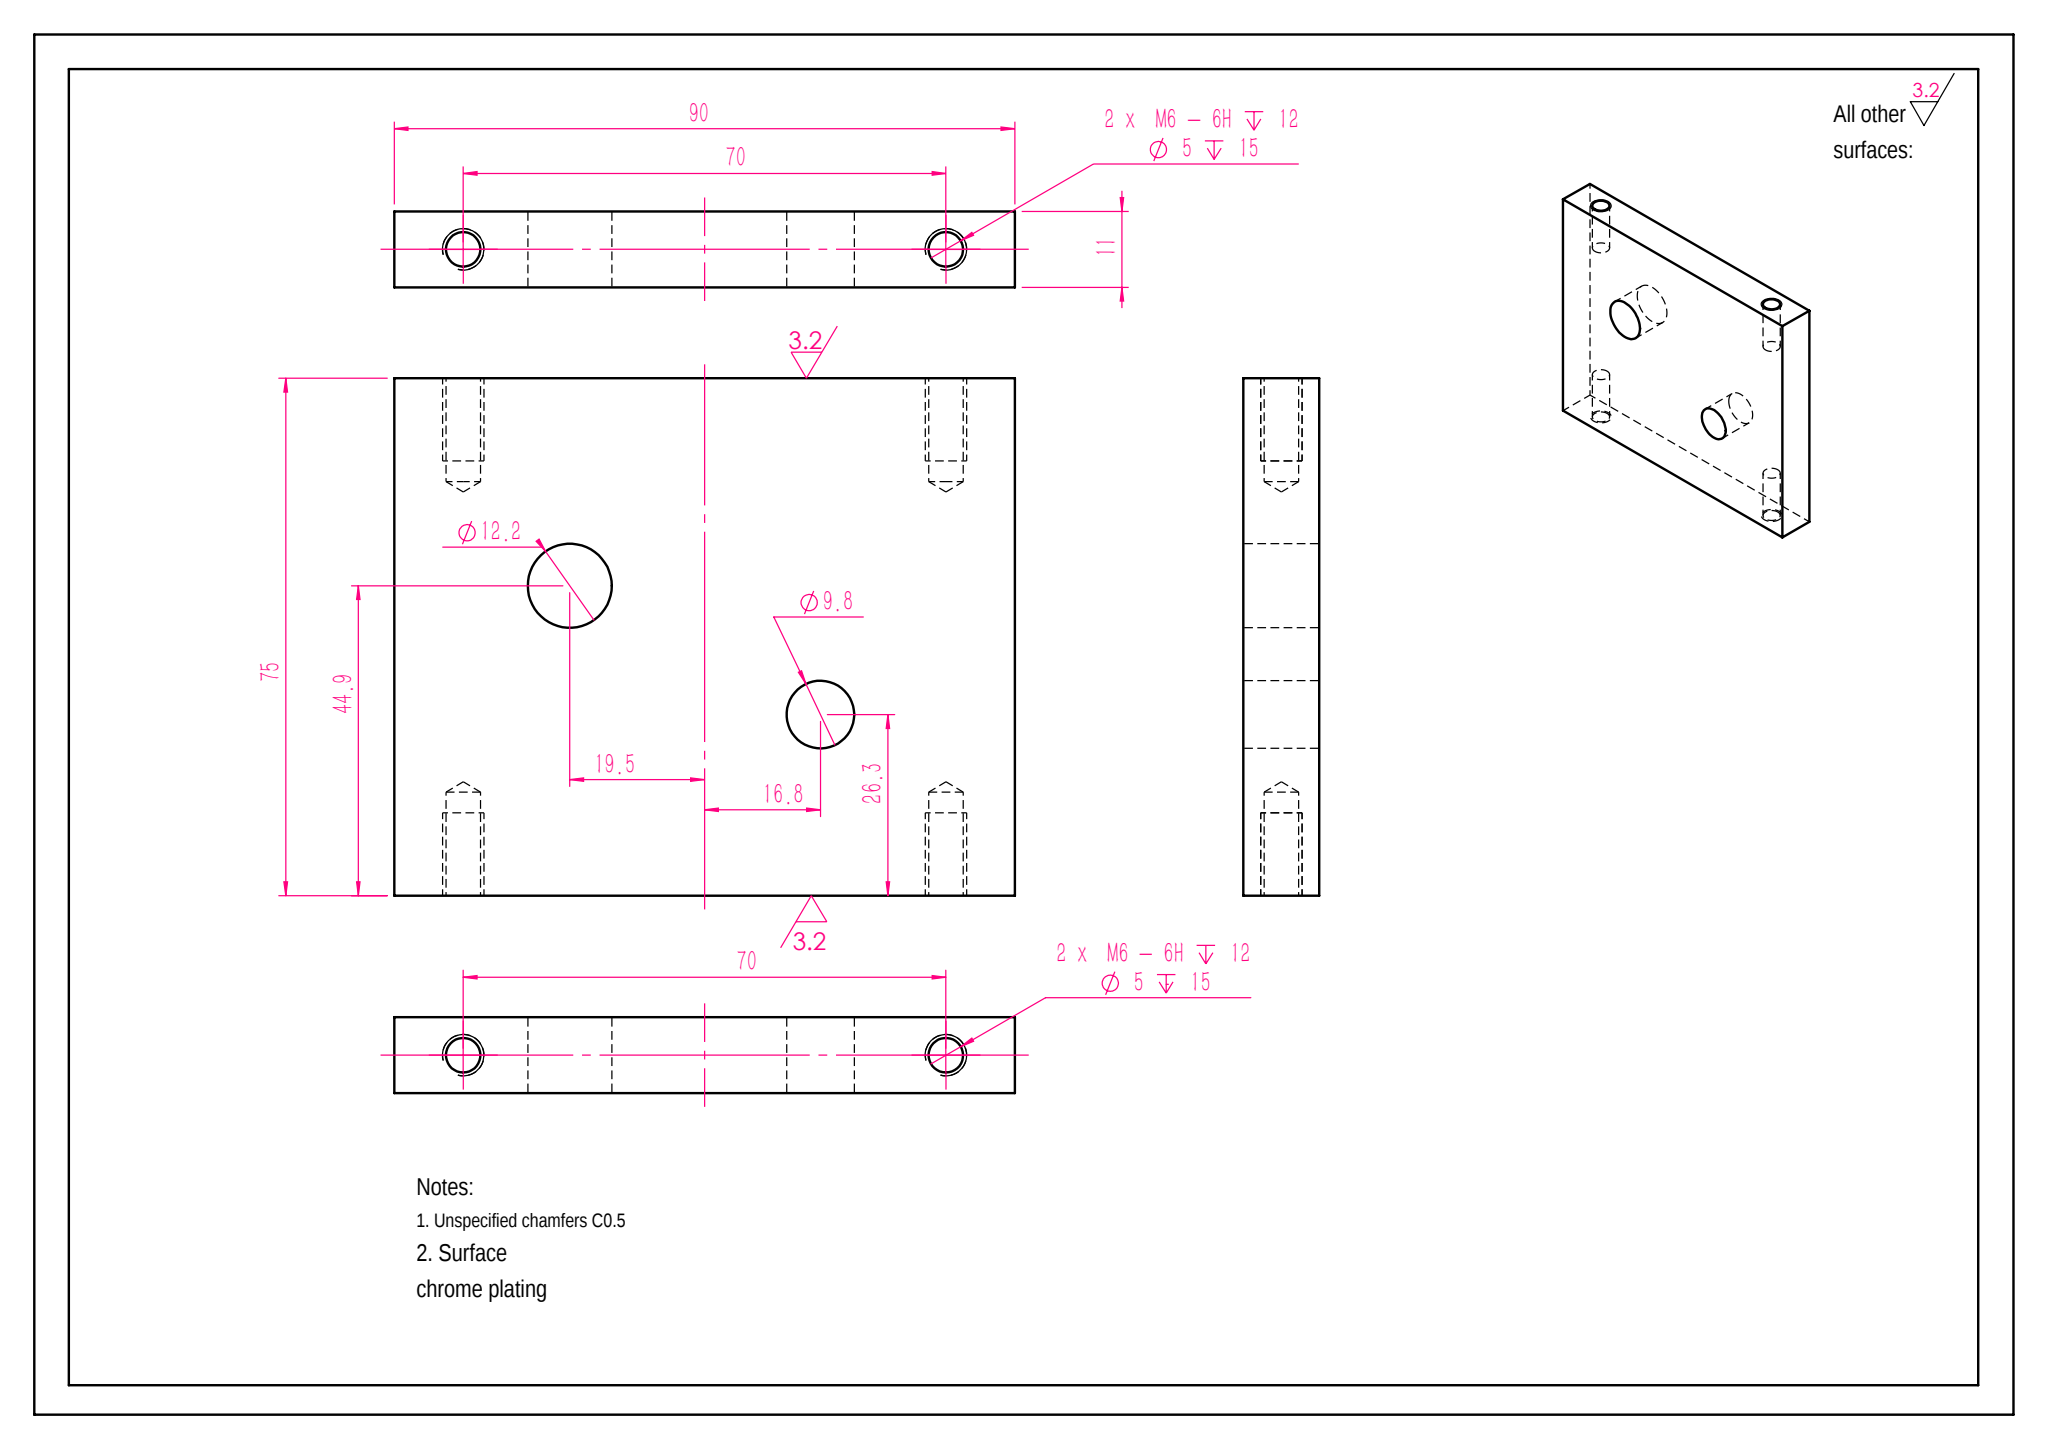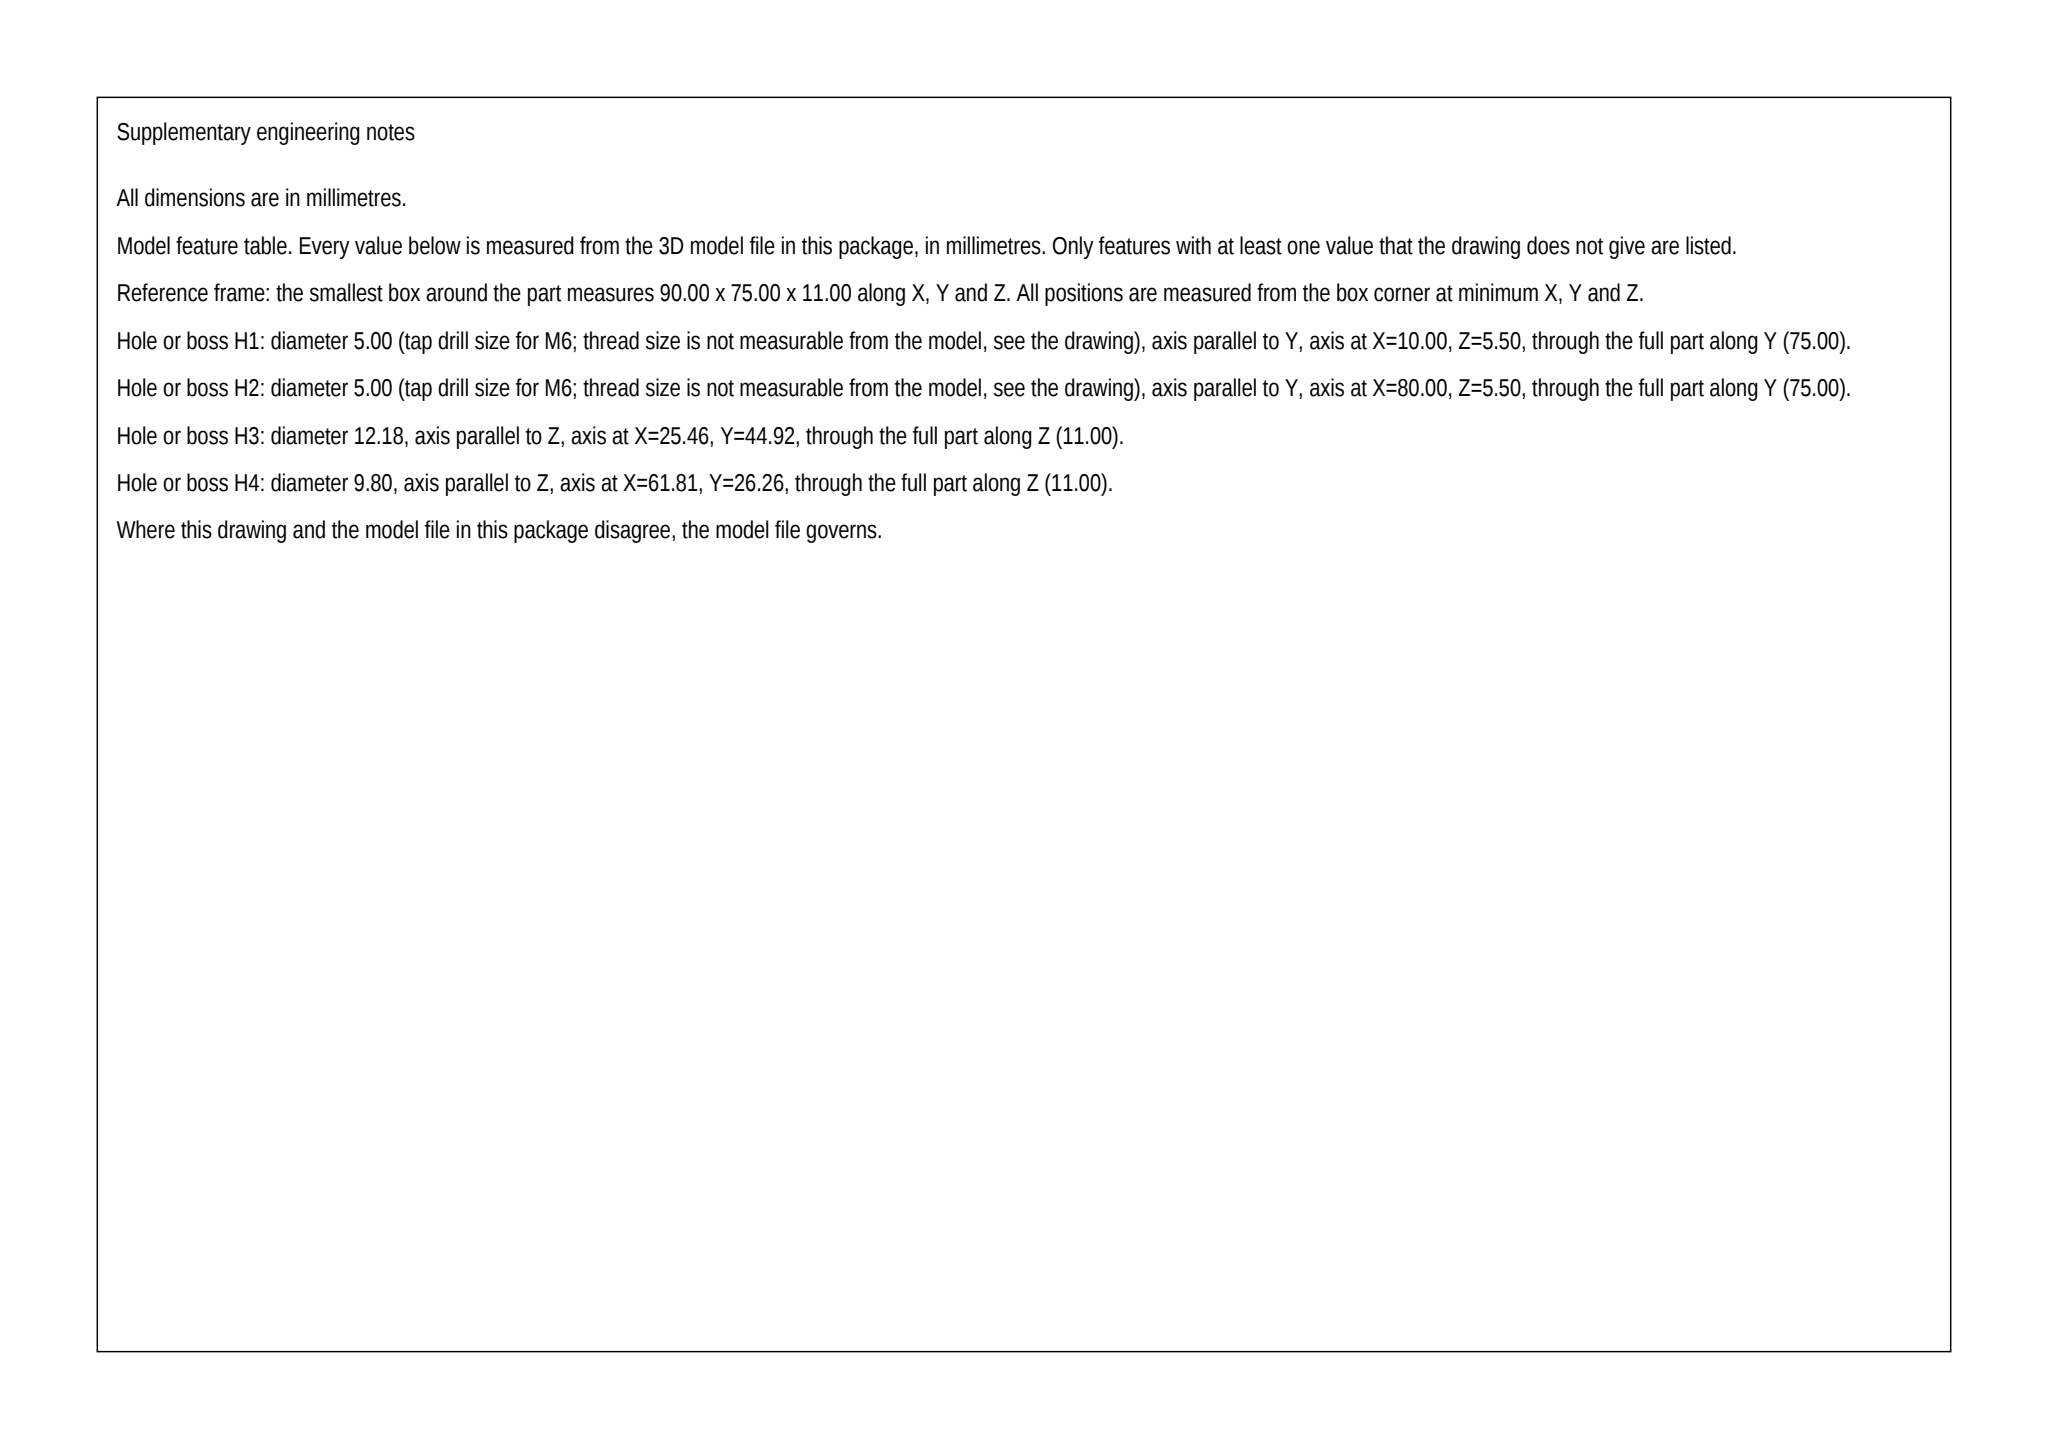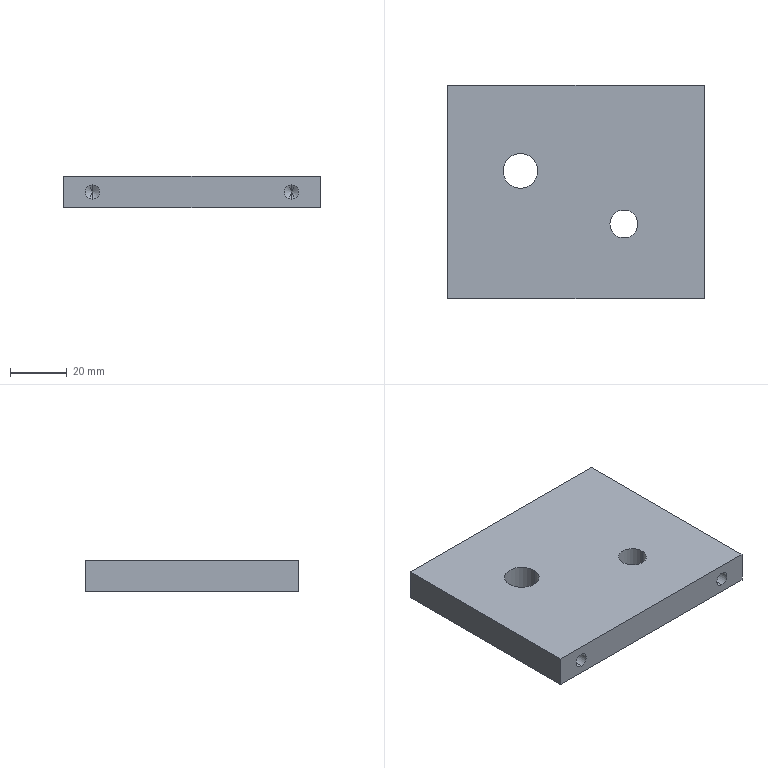Part | SolidWorks | mm | 1 solid | 26 faces | box 90 x 75 x 11 mm | volume 70920 mm3 | cylinder 12 | cone 8 | plane 6 | commonest cylinder face diameters 5 x8 12.178 x2 9.807 x2
build123d program:
from build123d import *

# Parameters (mm, degrees)
SKETCH1_W             = 90
SKETCH1_H             = 75
BOSS_EXTRUDE1_DEPTH   = 11
M6_TAPPED_HOLE1_D     = 5
M6_TAPPED_HOLE1_DEPTH = 15
M6_TAPPED_HOLE1_TIP   = 1.502
M6_TAPPED_HOLE2_D     = 5
M6_TAPPED_HOLE2_DEPTH = 15
M6_TAPPED_HOLE2_TIP   = 1.502
SKETCH6_R             = 6.089
SKETCH6_R_2           = 4.903
CUT_EXTRUDE1_DEPTH    = 80


with BuildPart() as part:
    # Sketch1 → Boss-Extrude1 (new body)
    with BuildSketch(Plane.XY):
        Rectangle(SKETCH1_W, SKETCH1_H)
    extrude(amount=BOSS_EXTRUDE1_DEPTH)

    # M6 Tapped Hole1
    with Locations(Plane(origin=(0, 37.5, 0), x_dir=(1, 0, 0), z_dir=(0, 1, 0))):
        with Locations((-35, -5.5), (35, -5.5)):
            Hole(M6_TAPPED_HOLE1_D / 2, depth=M6_TAPPED_HOLE1_DEPTH)
            with Locations((0, 0, -(M6_TAPPED_HOLE1_DEPTH + M6_TAPPED_HOLE1_TIP / 2))):  # 118° drill point
                Cone(0, M6_TAPPED_HOLE1_D / 2, M6_TAPPED_HOLE1_TIP, mode=Mode.SUBTRACT)

    # M6 Tapped Hole2
    with Locations(Plane(origin=(0, -37.5, 0), x_dir=(-1, 0, 0), z_dir=(0, -1, 0))):
        with Locations((35, -5.5), (-35, -5.5)):
            Hole(M6_TAPPED_HOLE2_D / 2, depth=M6_TAPPED_HOLE2_DEPTH)
            with Locations((0, 0, -(M6_TAPPED_HOLE2_DEPTH + M6_TAPPED_HOLE2_TIP / 2))):  # 118° drill point
                Cone(0, M6_TAPPED_HOLE2_D / 2, M6_TAPPED_HOLE2_TIP, mode=Mode.SUBTRACT)

    # Sketch6 → Cut-Extrude1 (cut)
    with BuildSketch(Plane.XY.offset(11)):
        with Locations((-19.538, 7.422)):
            Circle(SKETCH6_R)
        with Locations((16.809, -11.243)):
            Circle(SKETCH6_R_2)
    extrude(amount=-CUT_EXTRUDE1_DEPTH, mode=Mode.SUBTRACT)


solid = part.part
STEP:
#1=CARTESIAN_POINT('',(-13.449,7.422,0.));
#2=VERTEX_POINT('',#1);
#3=CARTESIAN_POINT('',(-25.627,7.422,0.));
#4=VERTEX_POINT('',#3);
#5=CARTESIAN_POINT('',(-19.538,7.422,0.));
#6=DIRECTION('',(0.,0.,-1.));
#7=DIRECTION('',(-1.,0.,0.));
#8=AXIS2_PLACEMENT_3D('',#5,#6,#7);
#9=CIRCLE('',#8,6.089);
#10=EDGE_CURVE('',#2,#4,#9,.T.);
#11=ORIENTED_EDGE('',*,*,#10,.T.);
#12=CARTESIAN_POINT('',(-25.627,7.422,11.));
#13=VERTEX_POINT('',#12);
#14=CARTESIAN_POINT('',(-25.627,7.422,-69.));
#15=DIRECTION('',(0.,0.,1.));
#16=VECTOR('',#15,1000.);
#17=LINE('',#14,#16);
#18=EDGE_CURVE('',#4,#13,#17,.T.);
#19=ORIENTED_EDGE('',*,*,#18,.T.);
#20=CARTESIAN_POINT('',(-13.449,7.422,11.));
#21=VERTEX_POINT('',#20);
#22=CARTESIAN_POINT('',(-19.538,7.422,11.));
#23=DIRECTION('',(0.,0.,1.));
#24=DIRECTION('',(1.,0.,0.));
#25=AXIS2_PLACEMENT_3D('',#22,#23,#24);
#26=CIRCLE('',#25,6.089);
#27=EDGE_CURVE('',#13,#21,#26,.T.);
#28=ORIENTED_EDGE('',*,*,#27,.T.);
#29=CARTESIAN_POINT('',(-13.449,7.422,-69.));
#30=DIRECTION('',(0.,0.,1.));
#31=VECTOR('',#30,1000.);
#32=LINE('',#29,#31);
#33=EDGE_CURVE('',#2,#21,#32,.T.);
#34=ORIENTED_EDGE('',*,*,#33,.F.);
#35=EDGE_LOOP('',(#11,#19,#28,#34));
#36=FACE_OUTER_BOUND('',#35,.T.);
#37=CARTESIAN_POINT('',(-19.538,7.422,-69.));
#38=DIRECTION('',(0.,0.,1.));
#39=DIRECTION('',(1.,0.,0.));
#40=AXIS2_PLACEMENT_3D('',#37,#38,#39);
#41=CYLINDRICAL_SURFACE('',#40,6.089);
#42=ADVANCED_FACE('',(#36),#41,.F.);
#43=CARTESIAN_POINT('',(21.713,-11.243,0.));
#44=VERTEX_POINT('',#43);
#45=CARTESIAN_POINT('',(11.906,-11.243,0.));
#46=VERTEX_POINT('',#45);
#47=CARTESIAN_POINT('',(16.809,-11.243,0.));
#48=DIRECTION('',(0.,0.,-1.));
#49=DIRECTION('',(-1.,0.,0.));
#50=AXIS2_PLACEMENT_3D('',#47,#48,#49);
#51=CIRCLE('',#50,4.903);
#52=EDGE_CURVE('',#44,#46,#51,.T.);
#53=ORIENTED_EDGE('',*,*,#52,.T.);
#54=CARTESIAN_POINT('',(11.906,-11.243,11.));
#55=VERTEX_POINT('',#54);
#56=CARTESIAN_POINT('',(11.906,-11.243,-69.));
#57=DIRECTION('',(0.,0.,1.));
#58=VECTOR('',#57,1000.);
#59=LINE('',#56,#58);
#60=EDGE_CURVE('',#46,#55,#59,.T.);
#61=ORIENTED_EDGE('',*,*,#60,.T.);
#62=CARTESIAN_POINT('',(21.713,-11.243,11.));
#63=VERTEX_POINT('',#62);
#64=CARTESIAN_POINT('',(16.809,-11.243,11.));
#65=DIRECTION('',(0.,0.,1.));
#66=DIRECTION('',(1.,0.,0.));
#67=AXIS2_PLACEMENT_3D('',#64,#65,#66);
#68=CIRCLE('',#67,4.903);
#69=EDGE_CURVE('',#55,#63,#68,.T.);
#70=ORIENTED_EDGE('',*,*,#69,.T.);
#71=CARTESIAN_POINT('',(21.713,-11.243,-69.));
#72=DIRECTION('',(0.,0.,1.));
#73=VECTOR('',#72,1000.);
#74=LINE('',#71,#73);
#75=EDGE_CURVE('',#44,#63,#74,.T.);
#76=ORIENTED_EDGE('',*,*,#75,.F.);
#77=EDGE_LOOP('',(#53,#61,#70,#76));
#78=FACE_OUTER_BOUND('',#77,.T.);
#79=CARTESIAN_POINT('',(16.809,-11.243,-69.));
#80=DIRECTION('',(0.,0.,1.));
#81=DIRECTION('',(1.,0.,0.));
#82=AXIS2_PLACEMENT_3D('',#79,#80,#81);
#83=CYLINDRICAL_SURFACE('',#82,4.903);
#84=ADVANCED_FACE('',(#78),#83,.F.);
#85=CARTESIAN_POINT('',(-35.,-22.5,8.));
#86=VERTEX_POINT('',#85);
#87=CARTESIAN_POINT('',(-35.,-22.5,3.));
#88=VERTEX_POINT('',#87);
#89=CARTESIAN_POINT('',(-35.,-22.5,5.5));
#90=DIRECTION('',(0.,-1.,0.));
#91=DIRECTION('',(0.,0.,-1.));
#92=AXIS2_PLACEMENT_3D('',#89,#90,#91);
#93=CIRCLE('',#92,2.5);
#94=EDGE_CURVE('',#86,#88,#93,.T.);
#95=ORIENTED_EDGE('',*,*,#94,.F.);
#96=CARTESIAN_POINT('',(-35.,-37.5,8.));
#97=VERTEX_POINT('',#96);
#98=CARTESIAN_POINT('',(-35.,-37.5,8.));
#99=DIRECTION('',(0.,-1.,0.));
#100=VECTOR('',#99,1000.);
#101=LINE('',#98,#100);
#102=EDGE_CURVE('',#86,#97,#101,.T.);
#103=ORIENTED_EDGE('',*,*,#102,.T.);
#104=CARTESIAN_POINT('',(-35.,-37.5,3.));
#105=VERTEX_POINT('',#104);
#106=CARTESIAN_POINT('',(-35.,-37.5,5.5));
#107=DIRECTION('',(0.,-1.,0.));
#108=DIRECTION('',(0.,0.,-1.));
#109=AXIS2_PLACEMENT_3D('',#106,#107,#108);
#110=CIRCLE('',#109,2.5);
#111=EDGE_CURVE('',#97,#105,#110,.T.);
#112=ORIENTED_EDGE('',*,*,#111,.T.);
#113=CARTESIAN_POINT('',(-35.,-37.5,3.));
#114=DIRECTION('',(0.,-1.,0.));
#115=VECTOR('',#114,1000.);
#116=LINE('',#113,#115);
#117=EDGE_CURVE('',#88,#105,#116,.T.);
#118=ORIENTED_EDGE('',*,*,#117,.F.);
#119=EDGE_LOOP('',(#95,#103,#112,#118));
#120=FACE_OUTER_BOUND('',#119,.T.);
#121=CARTESIAN_POINT('',(-35.,-37.5,5.5));
#122=DIRECTION('',(0.,-1.,0.));
#123=DIRECTION('',(0.,0.,-1.));
#124=AXIS2_PLACEMENT_3D('',#121,#122,#123);
#125=CYLINDRICAL_SURFACE('',#124,2.5);
#126=ADVANCED_FACE('',(#120),#125,.F.);
#127=CARTESIAN_POINT('',(-35.,-20.998,5.5));
#128=VERTEX_POINT('',#127);
#129=CARTESIAN_POINT('',(-35.,-22.5,3.));
#130=DIRECTION('',(0.,-0.515,-0.8572));
#131=VECTOR('',#130,1000.);
#132=LINE('',#129,#131);
#133=EDGE_CURVE('',#128,#88,#132,.T.);
#134=ORIENTED_EDGE('',*,*,#133,.F.);
#135=CARTESIAN_POINT('',(-35.,-22.5,8.));
#136=DIRECTION('',(0.,-0.515,0.8572));
#137=VECTOR('',#136,1000.);
#138=LINE('',#135,#137);
#139=EDGE_CURVE('',#128,#86,#138,.T.);
#140=ORIENTED_EDGE('',*,*,#139,.T.);
#141=ORIENTED_EDGE('',*,*,#94,.T.);
#142=EDGE_LOOP('',(#134,#140,#141));
#143=FACE_OUTER_BOUND('',#142,.T.);
#144=CARTESIAN_POINT('',(-35.,-22.5,5.5));
#145=DIRECTION('',(0.,-1.,0.));
#146=DIRECTION('',(0.,0.,-1.));
#147=AXIS2_PLACEMENT_3D('',#144,#145,#146);
#148=CONICAL_SURFACE('',#147,2.5,1.03);
#149=ADVANCED_FACE('',(#143),#148,.F.);
#150=CARTESIAN_POINT('',(35.,-22.5,8.));
#151=VERTEX_POINT('',#150);
#152=CARTESIAN_POINT('',(35.,-22.5,3.));
#153=VERTEX_POINT('',#152);
#154=CARTESIAN_POINT('',(35.,-22.5,5.5));
#155=DIRECTION('',(0.,-1.,0.));
#156=DIRECTION('',(0.,0.,-1.));
#157=AXIS2_PLACEMENT_3D('',#154,#155,#156);
#158=CIRCLE('',#157,2.5);
#159=EDGE_CURVE('',#151,#153,#158,.T.);
#160=ORIENTED_EDGE('',*,*,#159,.F.);
#161=CARTESIAN_POINT('',(35.,-37.5,8.));
#162=VERTEX_POINT('',#161);
#163=CARTESIAN_POINT('',(35.,-37.5,8.));
#164=DIRECTION('',(0.,-1.,0.));
#165=VECTOR('',#164,1000.);
#166=LINE('',#163,#165);
#167=EDGE_CURVE('',#151,#162,#166,.T.);
#168=ORIENTED_EDGE('',*,*,#167,.T.);
#169=CARTESIAN_POINT('',(35.,-37.5,3.));
#170=VERTEX_POINT('',#169);
#171=CARTESIAN_POINT('',(35.,-37.5,5.5));
#172=DIRECTION('',(0.,-1.,0.));
#173=DIRECTION('',(0.,0.,-1.));
#174=AXIS2_PLACEMENT_3D('',#171,#172,#173);
#175=CIRCLE('',#174,2.5);
#176=EDGE_CURVE('',#162,#170,#175,.T.);
#177=ORIENTED_EDGE('',*,*,#176,.T.);
#178=CARTESIAN_POINT('',(35.,-37.5,3.));
#179=DIRECTION('',(0.,-1.,0.));
#180=VECTOR('',#179,1000.);
#181=LINE('',#178,#180);
#182=EDGE_CURVE('',#153,#170,#181,.T.);
#183=ORIENTED_EDGE('',*,*,#182,.F.);
#184=EDGE_LOOP('',(#160,#168,#177,#183));
#185=FACE_OUTER_BOUND('',#184,.T.);
#186=CARTESIAN_POINT('',(35.,-37.5,5.5));
#187=DIRECTION('',(0.,-1.,0.));
#188=DIRECTION('',(0.,0.,-1.));
#189=AXIS2_PLACEMENT_3D('',#186,#187,#188);
#190=CYLINDRICAL_SURFACE('',#189,2.5);
#191=ADVANCED_FACE('',(#185),#190,.F.);
#192=CARTESIAN_POINT('',(35.,-20.998,5.5));
#193=VERTEX_POINT('',#192);
#194=CARTESIAN_POINT('',(35.,-22.5,3.));
#195=DIRECTION('',(0.,-0.515,-0.8572));
#196=VECTOR('',#195,1000.);
#197=LINE('',#194,#196);
#198=EDGE_CURVE('',#193,#153,#197,.T.);
#199=ORIENTED_EDGE('',*,*,#198,.F.);
#200=CARTESIAN_POINT('',(35.,-22.5,8.));
#201=DIRECTION('',(0.,-0.515,0.8572));
#202=VECTOR('',#201,1000.);
#203=LINE('',#200,#202);
#204=EDGE_CURVE('',#193,#151,#203,.T.);
#205=ORIENTED_EDGE('',*,*,#204,.T.);
#206=ORIENTED_EDGE('',*,*,#159,.T.);
#207=EDGE_LOOP('',(#199,#205,#206));
#208=FACE_OUTER_BOUND('',#207,.T.);
#209=CARTESIAN_POINT('',(35.,-22.5,5.5));
#210=DIRECTION('',(0.,-1.,0.));
#211=DIRECTION('',(0.,0.,-1.));
#212=AXIS2_PLACEMENT_3D('',#209,#210,#211);
#213=CONICAL_SURFACE('',#212,2.5,1.03);
#214=ADVANCED_FACE('',(#208),#213,.F.);
#215=CARTESIAN_POINT('',(-35.,22.5,3.));
#216=VERTEX_POINT('',#215);
#217=CARTESIAN_POINT('',(-35.,22.5,8.));
#218=VERTEX_POINT('',#217);
#219=CARTESIAN_POINT('',(-35.,22.5,5.5));
#220=DIRECTION('',(0.,1.,0.));
#221=DIRECTION('',(0.,0.,1.));
#222=AXIS2_PLACEMENT_3D('',#219,#220,#221);
#223=CIRCLE('',#222,2.5);
#224=EDGE_CURVE('',#216,#218,#223,.T.);
#225=ORIENTED_EDGE('',*,*,#224,.F.);
#226=CARTESIAN_POINT('',(-35.,37.5,3.));
#227=VERTEX_POINT('',#226);
#228=CARTESIAN_POINT('',(-35.,37.5,3.));
#229=DIRECTION('',(0.,1.,0.));
#230=VECTOR('',#229,1000.);
#231=LINE('',#228,#230);
#232=EDGE_CURVE('',#216,#227,#231,.T.);
#233=ORIENTED_EDGE('',*,*,#232,.T.);
#234=CARTESIAN_POINT('',(-35.,37.5,8.));
#235=VERTEX_POINT('',#234);
#236=CARTESIAN_POINT('',(-35.,37.5,5.5));
#237=DIRECTION('',(0.,1.,0.));
#238=DIRECTION('',(0.,0.,1.));
#239=AXIS2_PLACEMENT_3D('',#236,#237,#238);
#240=CIRCLE('',#239,2.5);
#241=EDGE_CURVE('',#227,#235,#240,.T.);
#242=ORIENTED_EDGE('',*,*,#241,.T.);
#243=CARTESIAN_POINT('',(-35.,37.5,8.));
#244=DIRECTION('',(0.,1.,0.));
#245=VECTOR('',#244,1000.);
#246=LINE('',#243,#245);
#247=EDGE_CURVE('',#218,#235,#246,.T.);
#248=ORIENTED_EDGE('',*,*,#247,.F.);
#249=EDGE_LOOP('',(#225,#233,#242,#248));
#250=FACE_OUTER_BOUND('',#249,.T.);
#251=CARTESIAN_POINT('',(-35.,37.5,5.5));
#252=DIRECTION('',(0.,1.,0.));
#253=DIRECTION('',(0.,0.,1.));
#254=AXIS2_PLACEMENT_3D('',#251,#252,#253);
#255=CYLINDRICAL_SURFACE('',#254,2.5);
#256=ADVANCED_FACE('',(#250),#255,.F.);
#257=CARTESIAN_POINT('',(-35.,20.998,5.5));
#258=VERTEX_POINT('',#257);
#259=CARTESIAN_POINT('',(-35.,22.5,8.));
#260=DIRECTION('',(0.,0.515,0.8572));
#261=VECTOR('',#260,1000.);
#262=LINE('',#259,#261);
#263=EDGE_CURVE('',#258,#218,#262,.T.);
#264=ORIENTED_EDGE('',*,*,#263,.F.);
#265=CARTESIAN_POINT('',(-35.,22.5,3.));
#266=DIRECTION('',(0.,0.515,-0.8572));
#267=VECTOR('',#266,1000.);
#268=LINE('',#265,#267);
#269=EDGE_CURVE('',#258,#216,#268,.T.);
#270=ORIENTED_EDGE('',*,*,#269,.T.);
#271=ORIENTED_EDGE('',*,*,#224,.T.);
#272=EDGE_LOOP('',(#264,#270,#271));
#273=FACE_OUTER_BOUND('',#272,.T.);
#274=CARTESIAN_POINT('',(-35.,22.5,5.5));
#275=DIRECTION('',(0.,1.,0.));
#276=DIRECTION('',(0.,0.,1.));
#277=AXIS2_PLACEMENT_3D('',#274,#275,#276);
#278=CONICAL_SURFACE('',#277,2.5,1.03);
#279=ADVANCED_FACE('',(#273),#278,.F.);
#280=CARTESIAN_POINT('',(35.,22.5,3.));
#281=VERTEX_POINT('',#280);
#282=CARTESIAN_POINT('',(35.,22.5,8.));
#283=VERTEX_POINT('',#282);
#284=CARTESIAN_POINT('',(35.,22.5,5.5));
#285=DIRECTION('',(0.,1.,0.));
#286=DIRECTION('',(0.,0.,1.));
#287=AXIS2_PLACEMENT_3D('',#284,#285,#286);
#288=CIRCLE('',#287,2.5);
#289=EDGE_CURVE('',#281,#283,#288,.T.);
#290=ORIENTED_EDGE('',*,*,#289,.F.);
#291=CARTESIAN_POINT('',(35.,37.5,3.));
#292=VERTEX_POINT('',#291);
#293=CARTESIAN_POINT('',(35.,37.5,3.));
#294=DIRECTION('',(0.,1.,0.));
#295=VECTOR('',#294,1000.);
#296=LINE('',#293,#295);
#297=EDGE_CURVE('',#281,#292,#296,.T.);
#298=ORIENTED_EDGE('',*,*,#297,.T.);
#299=CARTESIAN_POINT('',(35.,37.5,8.));
#300=VERTEX_POINT('',#299);
#301=CARTESIAN_POINT('',(35.,37.5,5.5));
#302=DIRECTION('',(0.,1.,0.));
#303=DIRECTION('',(0.,0.,1.));
#304=AXIS2_PLACEMENT_3D('',#301,#302,#303);
#305=CIRCLE('',#304,2.5);
#306=EDGE_CURVE('',#292,#300,#305,.T.);
#307=ORIENTED_EDGE('',*,*,#306,.T.);
#308=CARTESIAN_POINT('',(35.,37.5,8.));
#309=DIRECTION('',(0.,1.,0.));
#310=VECTOR('',#309,1000.);
#311=LINE('',#308,#310);
#312=EDGE_CURVE('',#283,#300,#311,.T.);
#313=ORIENTED_EDGE('',*,*,#312,.F.);
#314=EDGE_LOOP('',(#290,#298,#307,#313));
#315=FACE_OUTER_BOUND('',#314,.T.);
#316=CARTESIAN_POINT('',(35.,37.5,5.5));
#317=DIRECTION('',(0.,1.,0.));
#318=DIRECTION('',(0.,0.,1.));
#319=AXIS2_PLACEMENT_3D('',#316,#317,#318);
#320=CYLINDRICAL_SURFACE('',#319,2.5);
#321=ADVANCED_FACE('',(#315),#320,.F.);
#322=CARTESIAN_POINT('',(35.,20.998,5.5));
#323=VERTEX_POINT('',#322);
#324=CARTESIAN_POINT('',(35.,22.5,8.));
#325=DIRECTION('',(0.,0.515,0.8572));
#326=VECTOR('',#325,1000.);
#327=LINE('',#324,#326);
#328=EDGE_CURVE('',#323,#283,#327,.T.);
#329=ORIENTED_EDGE('',*,*,#328,.F.);
#330=CARTESIAN_POINT('',(35.,22.5,3.));
#331=DIRECTION('',(0.,0.515,-0.8572));
#332=VECTOR('',#331,1000.);
#333=LINE('',#330,#332);
#334=EDGE_CURVE('',#323,#281,#333,.T.);
#335=ORIENTED_EDGE('',*,*,#334,.T.);
#336=ORIENTED_EDGE('',*,*,#289,.T.);
#337=EDGE_LOOP('',(#329,#335,#336));
#338=FACE_OUTER_BOUND('',#337,.T.);
#339=CARTESIAN_POINT('',(35.,22.5,5.5));
#340=DIRECTION('',(0.,1.,0.));
#341=DIRECTION('',(0.,0.,1.));
#342=AXIS2_PLACEMENT_3D('',#339,#340,#341);
#343=CONICAL_SURFACE('',#342,2.5,1.03);
#344=ADVANCED_FACE('',(#338),#343,.F.);
#345=CARTESIAN_POINT('',(45.,-37.5,0.));
#346=VERTEX_POINT('',#345);
#347=CARTESIAN_POINT('',(45.,37.5,0.));
#348=VERTEX_POINT('',#347);
#349=CARTESIAN_POINT('',(45.,-37.5,0.));
#350=DIRECTION('',(0.,1.,0.));
#351=VECTOR('',#350,1000.);
#352=LINE('',#349,#351);
#353=EDGE_CURVE('',#346,#348,#352,.T.);
#354=ORIENTED_EDGE('',*,*,#353,.T.);
#355=CARTESIAN_POINT('',(45.,37.5,11.));
#356=VERTEX_POINT('',#355);
#357=CARTESIAN_POINT('',(45.,37.5,11.));
#358=DIRECTION('',(0.,0.,-1.));
#359=VECTOR('',#358,1000.);
#360=LINE('',#357,#359);
#361=EDGE_CURVE('',#356,#348,#360,.T.);
#362=ORIENTED_EDGE('',*,*,#361,.F.);
#363=CARTESIAN_POINT('',(45.,-37.5,11.));
#364=VERTEX_POINT('',#363);
#365=CARTESIAN_POINT('',(45.,-37.5,11.));
#366=DIRECTION('',(0.,1.,0.));
#367=VECTOR('',#366,1000.);
#368=LINE('',#365,#367);
#369=EDGE_CURVE('',#364,#356,#368,.T.);
#370=ORIENTED_EDGE('',*,*,#369,.F.);
#371=CARTESIAN_POINT('',(45.,-37.5,11.));
#372=DIRECTION('',(0.,0.,-1.));
#373=VECTOR('',#372,1000.);
#374=LINE('',#371,#373);
#375=EDGE_CURVE('',#364,#346,#374,.T.);
#376=ORIENTED_EDGE('',*,*,#375,.T.);
#377=EDGE_LOOP('',(#354,#362,#370,#376));
#378=FACE_OUTER_BOUND('',#377,.T.);
#379=CARTESIAN_POINT('',(45.,-37.5,11.));
#380=DIRECTION('',(-1.,0.,0.));
#381=DIRECTION('',(0.,0.,1.));
#382=AXIS2_PLACEMENT_3D('',#379,#380,#381);
#383=PLANE('',#382);
#384=ADVANCED_FACE('',(#378),#383,.F.);
#385=CARTESIAN_POINT('',(-35.,37.5,5.5));
#386=DIRECTION('',(0.,1.,0.));
#387=DIRECTION('',(0.,0.,1.));
#388=AXIS2_PLACEMENT_3D('',#385,#386,#387);
#389=CIRCLE('',#388,2.5);
#390=EDGE_CURVE('',#235,#227,#389,.T.);
#391=ORIENTED_EDGE('',*,*,#390,.F.);
#392=ORIENTED_EDGE('',*,*,#241,.F.);
#393=EDGE_LOOP('',(#391,#392));
#394=FACE_BOUND('',#393,.T.);
#395=CARTESIAN_POINT('',(35.,37.5,5.5));
#396=DIRECTION('',(0.,1.,0.));
#397=DIRECTION('',(0.,0.,1.));
#398=AXIS2_PLACEMENT_3D('',#395,#396,#397);
#399=CIRCLE('',#398,2.5);
#400=EDGE_CURVE('',#300,#292,#399,.T.);
#401=ORIENTED_EDGE('',*,*,#400,.F.);
#402=ORIENTED_EDGE('',*,*,#306,.F.);
#403=EDGE_LOOP('',(#401,#402));
#404=FACE_BOUND('',#403,.T.);
#405=CARTESIAN_POINT('',(-45.,37.5,0.));
#406=VERTEX_POINT('',#405);
#407=CARTESIAN_POINT('',(-45.,37.5,0.));
#408=DIRECTION('',(-1.,0.,0.));
#409=VECTOR('',#408,1000.);
#410=LINE('',#407,#409);
#411=EDGE_CURVE('',#348,#406,#410,.T.);
#412=ORIENTED_EDGE('',*,*,#411,.T.);
#413=CARTESIAN_POINT('',(-45.,37.5,11.));
#414=VERTEX_POINT('',#413);
#415=CARTESIAN_POINT('',(-45.,37.5,11.));
#416=DIRECTION('',(0.,0.,-1.));
#417=VECTOR('',#416,1000.);
#418=LINE('',#415,#417);
#419=EDGE_CURVE('',#414,#406,#418,.T.);
#420=ORIENTED_EDGE('',*,*,#419,.F.);
#421=CARTESIAN_POINT('',(-45.,37.5,11.));
#422=DIRECTION('',(-1.,0.,0.));
#423=VECTOR('',#422,1000.);
#424=LINE('',#421,#423);
#425=EDGE_CURVE('',#356,#414,#424,.T.);
#426=ORIENTED_EDGE('',*,*,#425,.F.);
#427=ORIENTED_EDGE('',*,*,#361,.T.);
#428=EDGE_LOOP('',(#412,#420,#426,#427));
#429=FACE_OUTER_BOUND('',#428,.T.);
#430=CARTESIAN_POINT('',(-45.,37.5,11.));
#431=DIRECTION('',(0.,-1.,0.));
#432=DIRECTION('',(0.,0.,-1.));
#433=AXIS2_PLACEMENT_3D('',#430,#431,#432);
#434=PLANE('',#433);
#435=ADVANCED_FACE('',(#394,#404,#429),#434,.F.);
#436=CARTESIAN_POINT('',(-45.,-37.5,0.));
#437=VERTEX_POINT('',#436);
#438=CARTESIAN_POINT('',(-45.,-37.5,0.));
#439=DIRECTION('',(0.,-1.,0.));
#440=VECTOR('',#439,1000.);
#441=LINE('',#438,#440);
#442=EDGE_CURVE('',#406,#437,#441,.T.);
#443=ORIENTED_EDGE('',*,*,#442,.T.);
#444=CARTESIAN_POINT('',(-45.,-37.5,11.));
#445=VERTEX_POINT('',#444);
#446=CARTESIAN_POINT('',(-45.,-37.5,11.));
#447=DIRECTION('',(0.,0.,-1.));
#448=VECTOR('',#447,1000.);
#449=LINE('',#446,#448);
#450=EDGE_CURVE('',#445,#437,#449,.T.);
#451=ORIENTED_EDGE('',*,*,#450,.F.);
#452=CARTESIAN_POINT('',(-45.,-37.5,11.));
#453=DIRECTION('',(0.,-1.,0.));
#454=VECTOR('',#453,1000.);
#455=LINE('',#452,#454);
#456=EDGE_CURVE('',#414,#445,#455,.T.);
#457=ORIENTED_EDGE('',*,*,#456,.F.);
#458=ORIENTED_EDGE('',*,*,#419,.T.);
#459=EDGE_LOOP('',(#443,#451,#457,#458));
#460=FACE_OUTER_BOUND('',#459,.T.);
#461=CARTESIAN_POINT('',(-45.,-37.5,11.));
#462=DIRECTION('',(1.,0.,0.));
#463=DIRECTION('',(0.,0.,-1.));
#464=AXIS2_PLACEMENT_3D('',#461,#462,#463);
#465=PLANE('',#464);
#466=ADVANCED_FACE('',(#460),#465,.F.);
#467=CARTESIAN_POINT('',(-35.,-37.5,5.5));
#468=DIRECTION('',(0.,-1.,0.));
#469=DIRECTION('',(0.,0.,-1.));
#470=AXIS2_PLACEMENT_3D('',#467,#468,#469);
#471=CIRCLE('',#470,2.5);
#472=EDGE_CURVE('',#105,#97,#471,.T.);
#473=ORIENTED_EDGE('',*,*,#472,.F.);
#474=ORIENTED_EDGE('',*,*,#111,.F.);
#475=EDGE_LOOP('',(#473,#474));
#476=FACE_BOUND('',#475,.T.);
#477=CARTESIAN_POINT('',(35.,-37.5,5.5));
#478=DIRECTION('',(0.,-1.,0.));
#479=DIRECTION('',(0.,0.,-1.));
#480=AXIS2_PLACEMENT_3D('',#477,#478,#479);
#481=CIRCLE('',#480,2.5);
#482=EDGE_CURVE('',#170,#162,#481,.T.);
#483=ORIENTED_EDGE('',*,*,#482,.F.);
#484=ORIENTED_EDGE('',*,*,#176,.F.);
#485=EDGE_LOOP('',(#483,#484));
#486=FACE_BOUND('',#485,.T.);
#487=CARTESIAN_POINT('',(-45.,-37.5,0.));
#488=DIRECTION('',(1.,0.,0.));
#489=VECTOR('',#488,1000.);
#490=LINE('',#487,#489);
#491=EDGE_CURVE('',#437,#346,#490,.T.);
#492=ORIENTED_EDGE('',*,*,#491,.T.);
#493=ORIENTED_EDGE('',*,*,#375,.F.);
#494=CARTESIAN_POINT('',(-45.,-37.5,11.));
#495=DIRECTION('',(1.,0.,0.));
#496=VECTOR('',#495,1000.);
#497=LINE('',#494,#496);
#498=EDGE_CURVE('',#445,#364,#497,.T.);
#499=ORIENTED_EDGE('',*,*,#498,.F.);
#500=ORIENTED_EDGE('',*,*,#450,.T.);
#501=EDGE_LOOP('',(#492,#493,#499,#500));
#502=FACE_OUTER_BOUND('',#501,.T.);
#503=CARTESIAN_POINT('',(-45.,-37.5,11.));
#504=DIRECTION('',(0.,1.,0.));
#505=DIRECTION('',(0.,0.,1.));
#506=AXIS2_PLACEMENT_3D('',#503,#504,#505);
#507=PLANE('',#506);
#508=ADVANCED_FACE('',(#476,#486,#502),#507,.F.);
#509=CARTESIAN_POINT('',(-19.538,7.422,11.));
#510=DIRECTION('',(0.,0.,1.));
#511=DIRECTION('',(1.,0.,0.));
#512=AXIS2_PLACEMENT_3D('',#509,#510,#511);
#513=CIRCLE('',#512,6.089);
#514=EDGE_CURVE('',#21,#13,#513,.T.);
#515=ORIENTED_EDGE('',*,*,#514,.F.);
#516=ORIENTED_EDGE('',*,*,#27,.F.);
#517=EDGE_LOOP('',(#515,#516));
#518=FACE_BOUND('',#517,.T.);
#519=CARTESIAN_POINT('',(16.809,-11.243,11.));
#520=DIRECTION('',(0.,0.,1.));
#521=DIRECTION('',(1.,0.,0.));
#522=AXIS2_PLACEMENT_3D('',#519,#520,#521);
#523=CIRCLE('',#522,4.903);
#524=EDGE_CURVE('',#63,#55,#523,.T.);
#525=ORIENTED_EDGE('',*,*,#524,.F.);
#526=ORIENTED_EDGE('',*,*,#69,.F.);
#527=EDGE_LOOP('',(#525,#526));
#528=FACE_BOUND('',#527,.T.);
#529=ORIENTED_EDGE('',*,*,#369,.T.);
#530=ORIENTED_EDGE('',*,*,#425,.T.);
#531=ORIENTED_EDGE('',*,*,#456,.T.);
#532=ORIENTED_EDGE('',*,*,#498,.T.);
#533=EDGE_LOOP('',(#529,#530,#531,#532));
#534=FACE_OUTER_BOUND('',#533,.T.);
#535=CARTESIAN_POINT('',(0.,0.,11.));
#536=DIRECTION('',(0.,0.,-1.));
#537=DIRECTION('',(-1.,0.,0.));
#538=AXIS2_PLACEMENT_3D('',#535,#536,#537);
#539=PLANE('',#538);
#540=ADVANCED_FACE('',(#518,#528,#534),#539,.F.);
#541=ORIENTED_EDGE('',*,*,#10,.F.);
#542=CARTESIAN_POINT('',(-19.538,7.422,0.));
#543=DIRECTION('',(0.,0.,-1.));
#544=DIRECTION('',(-1.,0.,0.));
#545=AXIS2_PLACEMENT_3D('',#542,#543,#544);
#546=CIRCLE('',#545,6.089);
#547=EDGE_CURVE('',#4,#2,#546,.T.);
#548=ORIENTED_EDGE('',*,*,#547,.F.);
#549=EDGE_LOOP('',(#541,#548));
#550=FACE_BOUND('',#549,.T.);
#551=ORIENTED_EDGE('',*,*,#52,.F.);
#552=CARTESIAN_POINT('',(16.809,-11.243,0.));
#553=DIRECTION('',(0.,0.,-1.));
#554=DIRECTION('',(-1.,0.,0.));
#555=AXIS2_PLACEMENT_3D('',#552,#553,#554);
#556=CIRCLE('',#555,4.903);
#557=EDGE_CURVE('',#46,#44,#556,.T.);
#558=ORIENTED_EDGE('',*,*,#557,.F.);
#559=EDGE_LOOP('',(#551,#558));
#560=FACE_BOUND('',#559,.T.);
#561=ORIENTED_EDGE('',*,*,#353,.F.);
#562=ORIENTED_EDGE('',*,*,#491,.F.);
#563=ORIENTED_EDGE('',*,*,#442,.F.);
#564=ORIENTED_EDGE('',*,*,#411,.F.);
#565=EDGE_LOOP('',(#561,#562,#563,#564));
#566=FACE_OUTER_BOUND('',#565,.T.);
#567=CARTESIAN_POINT('',(0.,0.,0.));
#568=DIRECTION('',(0.,0.,-1.));
#569=DIRECTION('',(-1.,0.,0.));
#570=AXIS2_PLACEMENT_3D('',#567,#568,#569);
#571=PLANE('',#570);
#572=ADVANCED_FACE('',(#550,#560,#566),#571,.T.);
#573=ORIENTED_EDGE('',*,*,#334,.F.);
#574=ORIENTED_EDGE('',*,*,#328,.T.);
#575=CARTESIAN_POINT('',(35.,22.5,5.5));
#576=DIRECTION('',(0.,1.,0.));
#577=DIRECTION('',(0.,0.,1.));
#578=AXIS2_PLACEMENT_3D('',#575,#576,#577);
#579=CIRCLE('',#578,2.5);
#580=EDGE_CURVE('',#283,#281,#579,.T.);
#581=ORIENTED_EDGE('',*,*,#580,.T.);
#582=EDGE_LOOP('',(#573,#574,#581));
#583=FACE_OUTER_BOUND('',#582,.T.);
#584=CARTESIAN_POINT('',(35.,22.5,5.5));
#585=DIRECTION('',(0.,1.,0.));
#586=DIRECTION('',(0.,0.,1.));
#587=AXIS2_PLACEMENT_3D('',#584,#585,#586);
#588=CONICAL_SURFACE('',#587,2.5,1.03);
#589=ADVANCED_FACE('',(#583),#588,.F.);
#590=ORIENTED_EDGE('',*,*,#297,.F.);
#591=ORIENTED_EDGE('',*,*,#580,.F.);
#592=ORIENTED_EDGE('',*,*,#312,.T.);
#593=ORIENTED_EDGE('',*,*,#400,.T.);
#594=EDGE_LOOP('',(#590,#591,#592,#593));
#595=FACE_OUTER_BOUND('',#594,.T.);
#596=CARTESIAN_POINT('',(35.,37.5,5.5));
#597=DIRECTION('',(0.,1.,0.));
#598=DIRECTION('',(0.,0.,1.));
#599=AXIS2_PLACEMENT_3D('',#596,#597,#598);
#600=CYLINDRICAL_SURFACE('',#599,2.5);
#601=ADVANCED_FACE('',(#595),#600,.F.);
#602=ORIENTED_EDGE('',*,*,#269,.F.);
#603=ORIENTED_EDGE('',*,*,#263,.T.);
#604=CARTESIAN_POINT('',(-35.,22.5,5.5));
#605=DIRECTION('',(0.,1.,0.));
#606=DIRECTION('',(0.,0.,1.));
#607=AXIS2_PLACEMENT_3D('',#604,#605,#606);
#608=CIRCLE('',#607,2.5);
#609=EDGE_CURVE('',#218,#216,#608,.T.);
#610=ORIENTED_EDGE('',*,*,#609,.T.);
#611=EDGE_LOOP('',(#602,#603,#610));
#612=FACE_OUTER_BOUND('',#611,.T.);
#613=CARTESIAN_POINT('',(-35.,22.5,5.5));
#614=DIRECTION('',(0.,1.,0.));
#615=DIRECTION('',(0.,0.,1.));
#616=AXIS2_PLACEMENT_3D('',#613,#614,#615);
#617=CONICAL_SURFACE('',#616,2.5,1.03);
#618=ADVANCED_FACE('',(#612),#617,.F.);
#619=ORIENTED_EDGE('',*,*,#232,.F.);
#620=ORIENTED_EDGE('',*,*,#609,.F.);
#621=ORIENTED_EDGE('',*,*,#247,.T.);
#622=ORIENTED_EDGE('',*,*,#390,.T.);
#623=EDGE_LOOP('',(#619,#620,#621,#622));
#624=FACE_OUTER_BOUND('',#623,.T.);
#625=CARTESIAN_POINT('',(-35.,37.5,5.5));
#626=DIRECTION('',(0.,1.,0.));
#627=DIRECTION('',(0.,0.,1.));
#628=AXIS2_PLACEMENT_3D('',#625,#626,#627);
#629=CYLINDRICAL_SURFACE('',#628,2.5);
#630=ADVANCED_FACE('',(#624),#629,.F.);
#631=ORIENTED_EDGE('',*,*,#204,.F.);
#632=ORIENTED_EDGE('',*,*,#198,.T.);
#633=CARTESIAN_POINT('',(35.,-22.5,5.5));
#634=DIRECTION('',(0.,-1.,0.));
#635=DIRECTION('',(0.,0.,-1.));
#636=AXIS2_PLACEMENT_3D('',#633,#634,#635);
#637=CIRCLE('',#636,2.5);
#638=EDGE_CURVE('',#153,#151,#637,.T.);
#639=ORIENTED_EDGE('',*,*,#638,.T.);
#640=EDGE_LOOP('',(#631,#632,#639));
#641=FACE_OUTER_BOUND('',#640,.T.);
#642=CARTESIAN_POINT('',(35.,-22.5,5.5));
#643=DIRECTION('',(0.,-1.,0.));
#644=DIRECTION('',(0.,0.,-1.));
#645=AXIS2_PLACEMENT_3D('',#642,#643,#644);
#646=CONICAL_SURFACE('',#645,2.5,1.03);
#647=ADVANCED_FACE('',(#641),#646,.F.);
#648=ORIENTED_EDGE('',*,*,#167,.F.);
#649=ORIENTED_EDGE('',*,*,#638,.F.);
#650=ORIENTED_EDGE('',*,*,#182,.T.);
#651=ORIENTED_EDGE('',*,*,#482,.T.);
#652=EDGE_LOOP('',(#648,#649,#650,#651));
#653=FACE_OUTER_BOUND('',#652,.T.);
#654=CARTESIAN_POINT('',(35.,-37.5,5.5));
#655=DIRECTION('',(0.,-1.,0.));
#656=DIRECTION('',(0.,0.,-1.));
#657=AXIS2_PLACEMENT_3D('',#654,#655,#656);
#658=CYLINDRICAL_SURFACE('',#657,2.5);
#659=ADVANCED_FACE('',(#653),#658,.F.);
#660=ORIENTED_EDGE('',*,*,#139,.F.);
#661=ORIENTED_EDGE('',*,*,#133,.T.);
#662=CARTESIAN_POINT('',(-35.,-22.5,5.5));
#663=DIRECTION('',(0.,-1.,0.));
#664=DIRECTION('',(0.,0.,-1.));
#665=AXIS2_PLACEMENT_3D('',#662,#663,#664);
#666=CIRCLE('',#665,2.5);
#667=EDGE_CURVE('',#88,#86,#666,.T.);
#668=ORIENTED_EDGE('',*,*,#667,.T.);
#669=EDGE_LOOP('',(#660,#661,#668));
#670=FACE_OUTER_BOUND('',#669,.T.);
#671=CARTESIAN_POINT('',(-35.,-22.5,5.5));
#672=DIRECTION('',(0.,-1.,0.));
#673=DIRECTION('',(0.,0.,-1.));
#674=AXIS2_PLACEMENT_3D('',#671,#672,#673);
#675=CONICAL_SURFACE('',#674,2.5,1.03);
#676=ADVANCED_FACE('',(#670),#675,.F.);
#677=ORIENTED_EDGE('',*,*,#102,.F.);
#678=ORIENTED_EDGE('',*,*,#667,.F.);
#679=ORIENTED_EDGE('',*,*,#117,.T.);
#680=ORIENTED_EDGE('',*,*,#472,.T.);
#681=EDGE_LOOP('',(#677,#678,#679,#680));
#682=FACE_OUTER_BOUND('',#681,.T.);
#683=CARTESIAN_POINT('',(-35.,-37.5,5.5));
#684=DIRECTION('',(0.,-1.,0.));
#685=DIRECTION('',(0.,0.,-1.));
#686=AXIS2_PLACEMENT_3D('',#683,#684,#685);
#687=CYLINDRICAL_SURFACE('',#686,2.5);
#688=ADVANCED_FACE('',(#682),#687,.F.);
#689=ORIENTED_EDGE('',*,*,#60,.F.);
#690=ORIENTED_EDGE('',*,*,#557,.T.);
#691=ORIENTED_EDGE('',*,*,#75,.T.);
#692=ORIENTED_EDGE('',*,*,#524,.T.);
#693=EDGE_LOOP('',(#689,#690,#691,#692));
#694=FACE_OUTER_BOUND('',#693,.T.);
#695=CARTESIAN_POINT('',(16.809,-11.243,-69.));
#696=DIRECTION('',(0.,0.,1.));
#697=DIRECTION('',(1.,0.,0.));
#698=AXIS2_PLACEMENT_3D('',#695,#696,#697);
#699=CYLINDRICAL_SURFACE('',#698,4.903);
#700=ADVANCED_FACE('',(#694),#699,.F.);
#701=ORIENTED_EDGE('',*,*,#18,.F.);
#702=ORIENTED_EDGE('',*,*,#547,.T.);
#703=ORIENTED_EDGE('',*,*,#33,.T.);
#704=ORIENTED_EDGE('',*,*,#514,.T.);
#705=EDGE_LOOP('',(#701,#702,#703,#704));
#706=FACE_OUTER_BOUND('',#705,.T.);
#707=CARTESIAN_POINT('',(-19.538,7.422,-69.));
#708=DIRECTION('',(0.,0.,1.));
#709=DIRECTION('',(1.,0.,0.));
#710=AXIS2_PLACEMENT_3D('',#707,#708,#709);
#711=CYLINDRICAL_SURFACE('',#710,6.089);
#712=ADVANCED_FACE('',(#706),#711,.F.);
#713=CLOSED_SHELL('',(#42,#84,#126,#149,#191,#214,#256,#279,#321,#344,#384,#435,#466,#508,#540,#572,#589,#601,#618,#630,#647,#659,#676,#688,#700,#712));
#714=MANIFOLD_SOLID_BREP('',#713);
#715=CARTESIAN_POINT('',(0.,0.,0.));
#716=DIRECTION('',(0.,0.,1.));
#717=DIRECTION('',(1.,0.,0.));
#718=AXIS2_PLACEMENT_3D('',#715,#716,#717);
#719=(LENGTH_UNIT()NAMED_UNIT(*)SI_UNIT(.MILLI.,.METRE.));
#720=UNCERTAINTY_MEASURE_WITH_UNIT(LENGTH_MEASURE(0.00001),#719,'','');
#721=(NAMED_UNIT(*)PLANE_ANGLE_UNIT()SI_UNIT($,.RADIAN.));
#722=(NAMED_UNIT(*)SI_UNIT($,.STERADIAN.)SOLID_ANGLE_UNIT());
#723=(GEOMETRIC_REPRESENTATION_CONTEXT(3)GLOBAL_UNCERTAINTY_ASSIGNED_CONTEXT((#720))GLOBAL_UNIT_ASSIGNED_CONTEXT((#719,#721,#722))REPRESENTATION_CONTEXT('',''));
#724=ADVANCED_BREP_SHAPE_REPRESENTATION('',(#714,#718),#723);